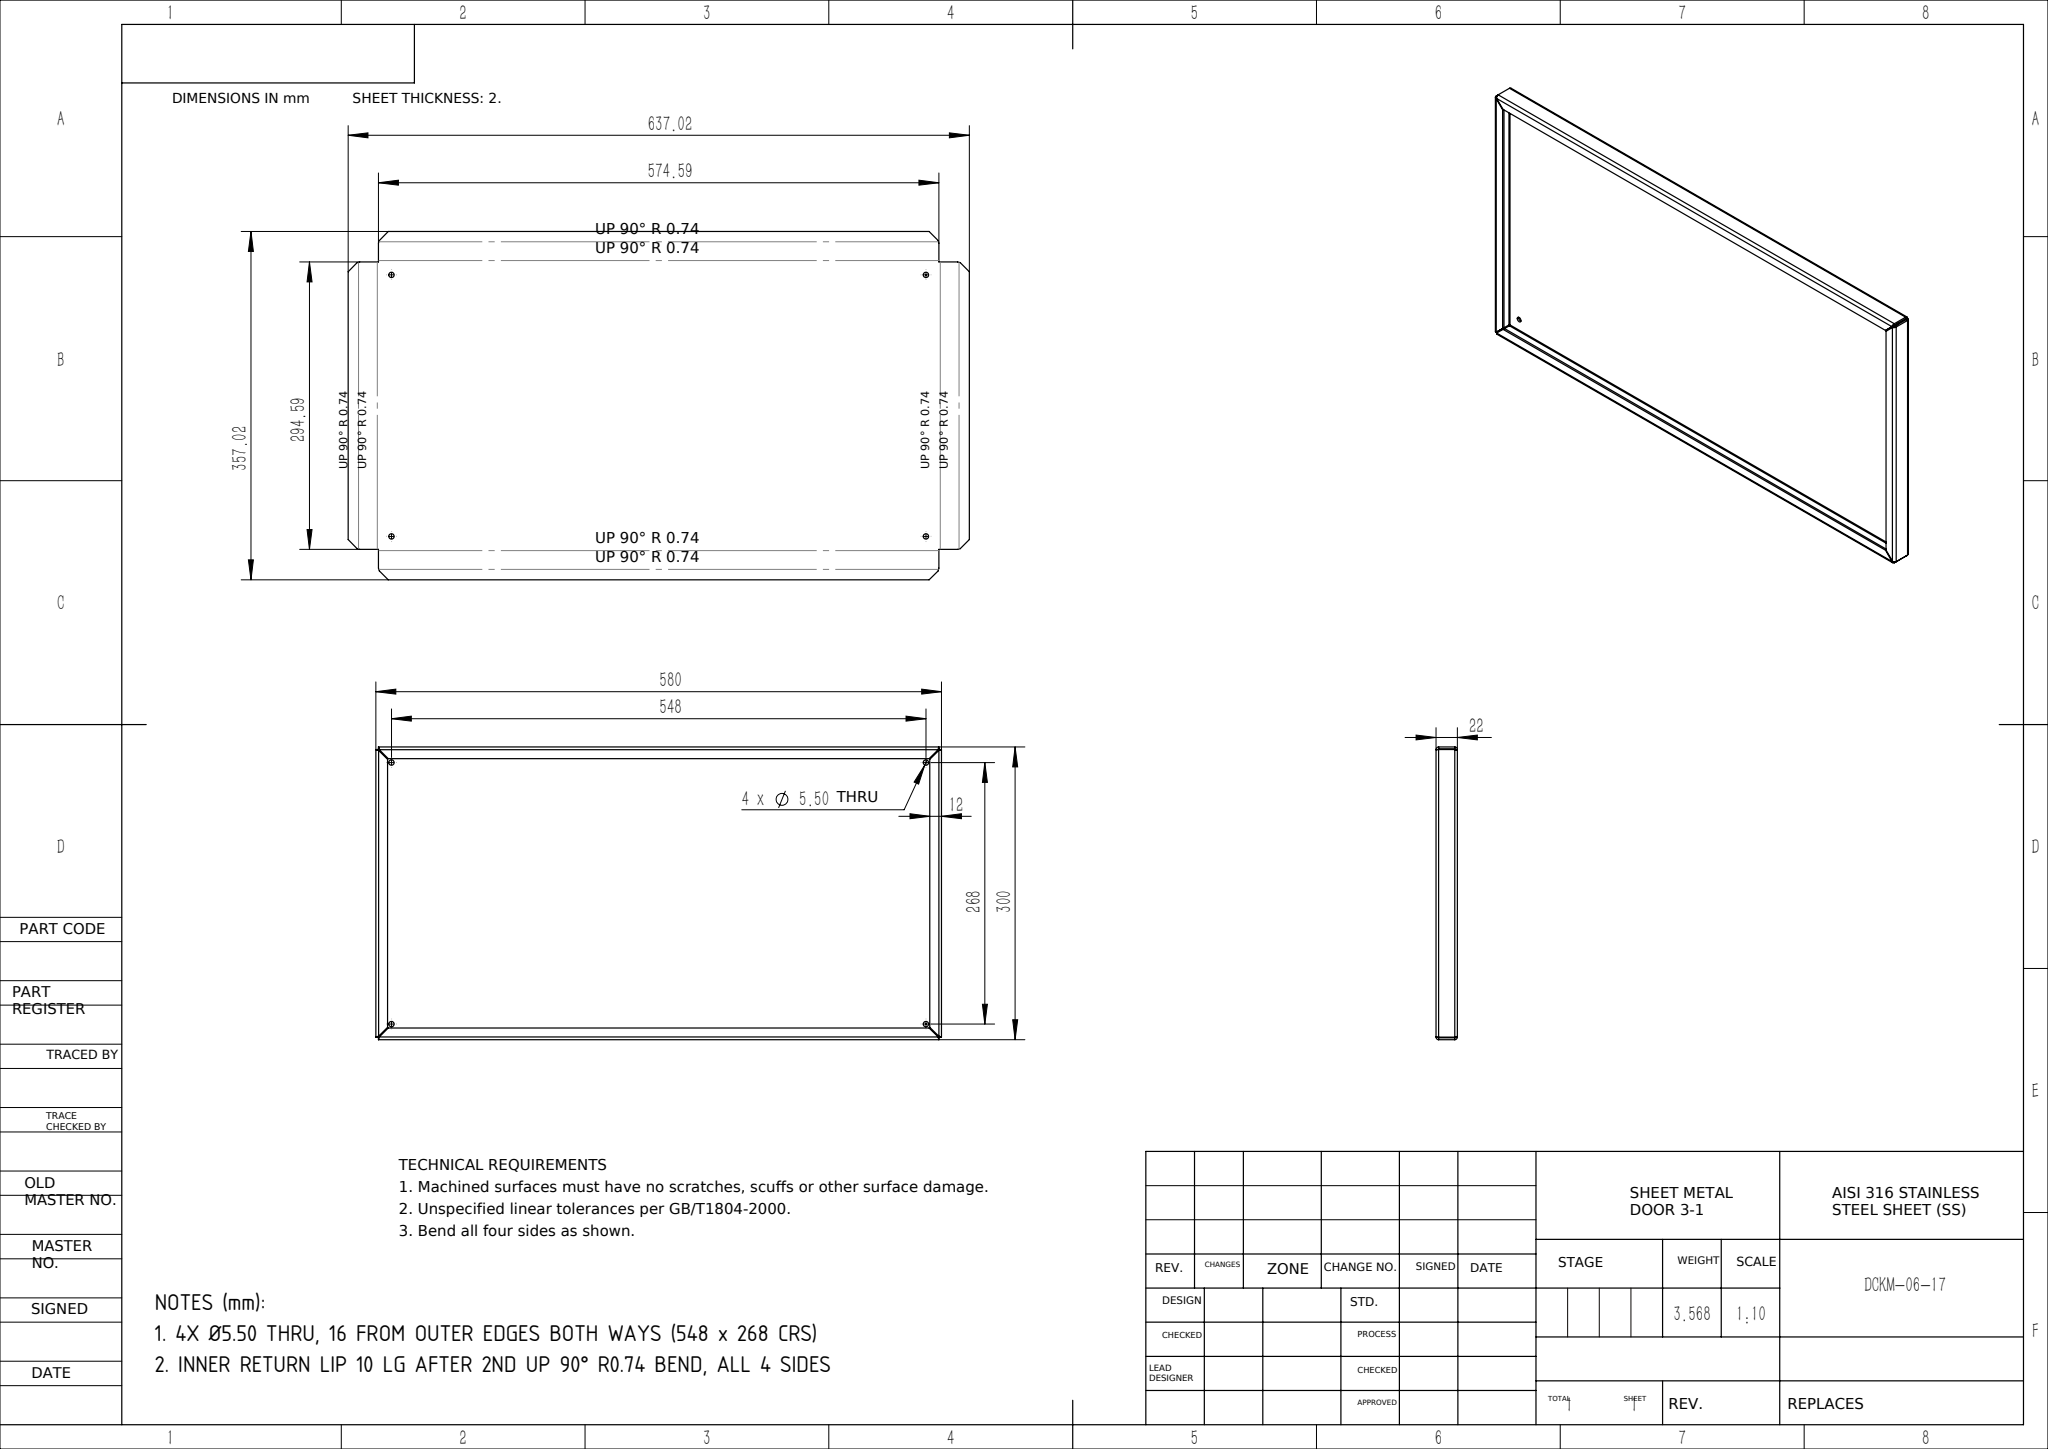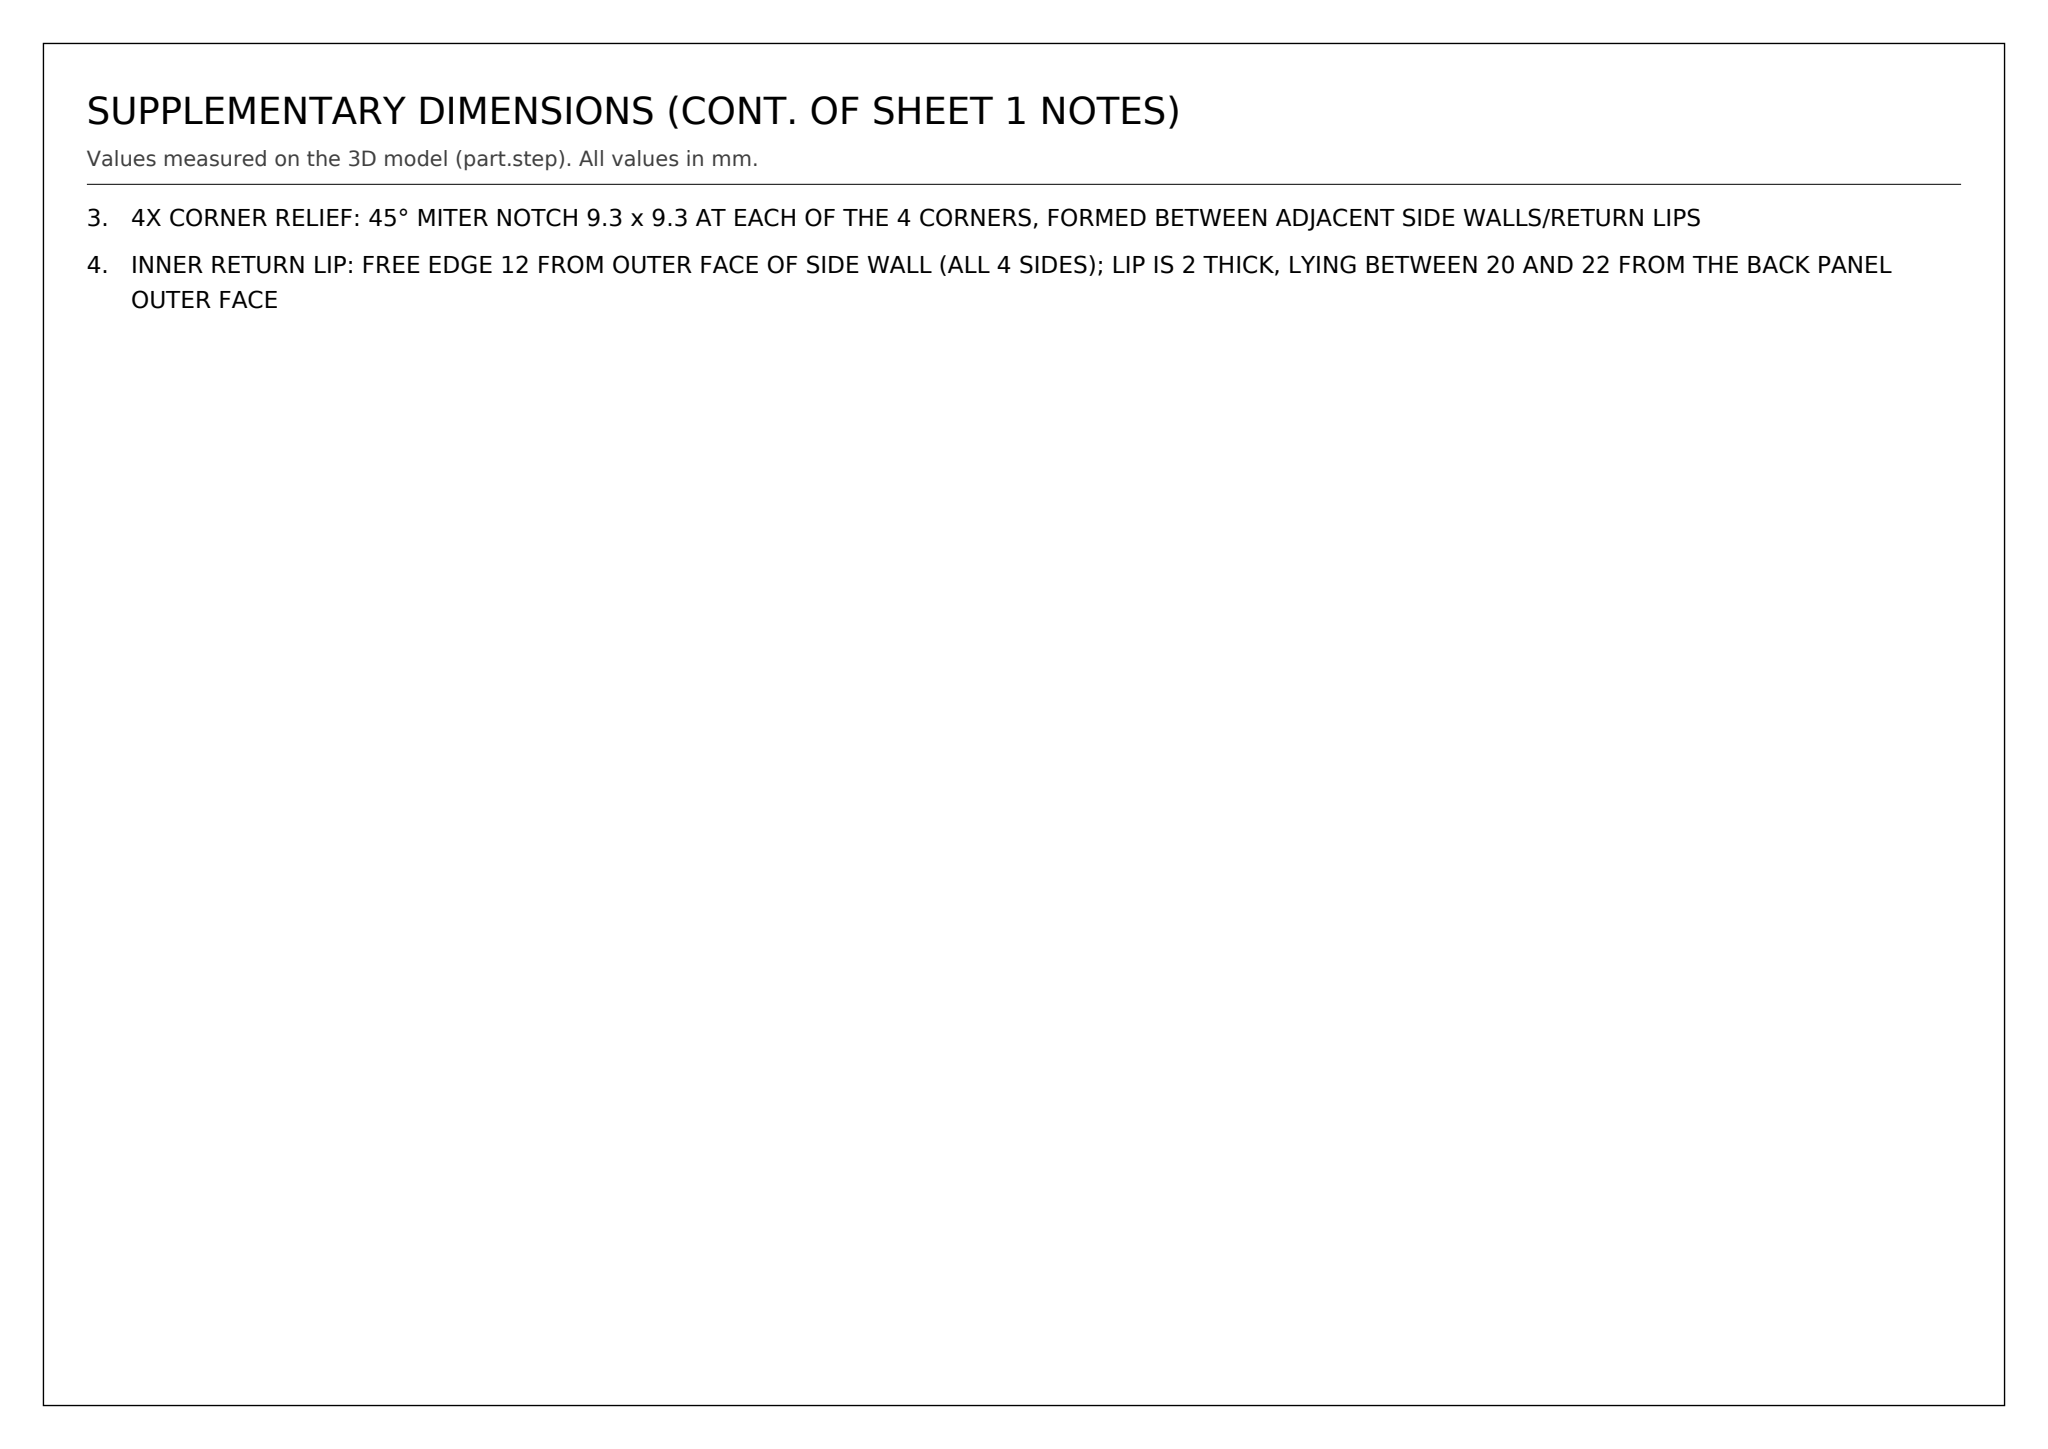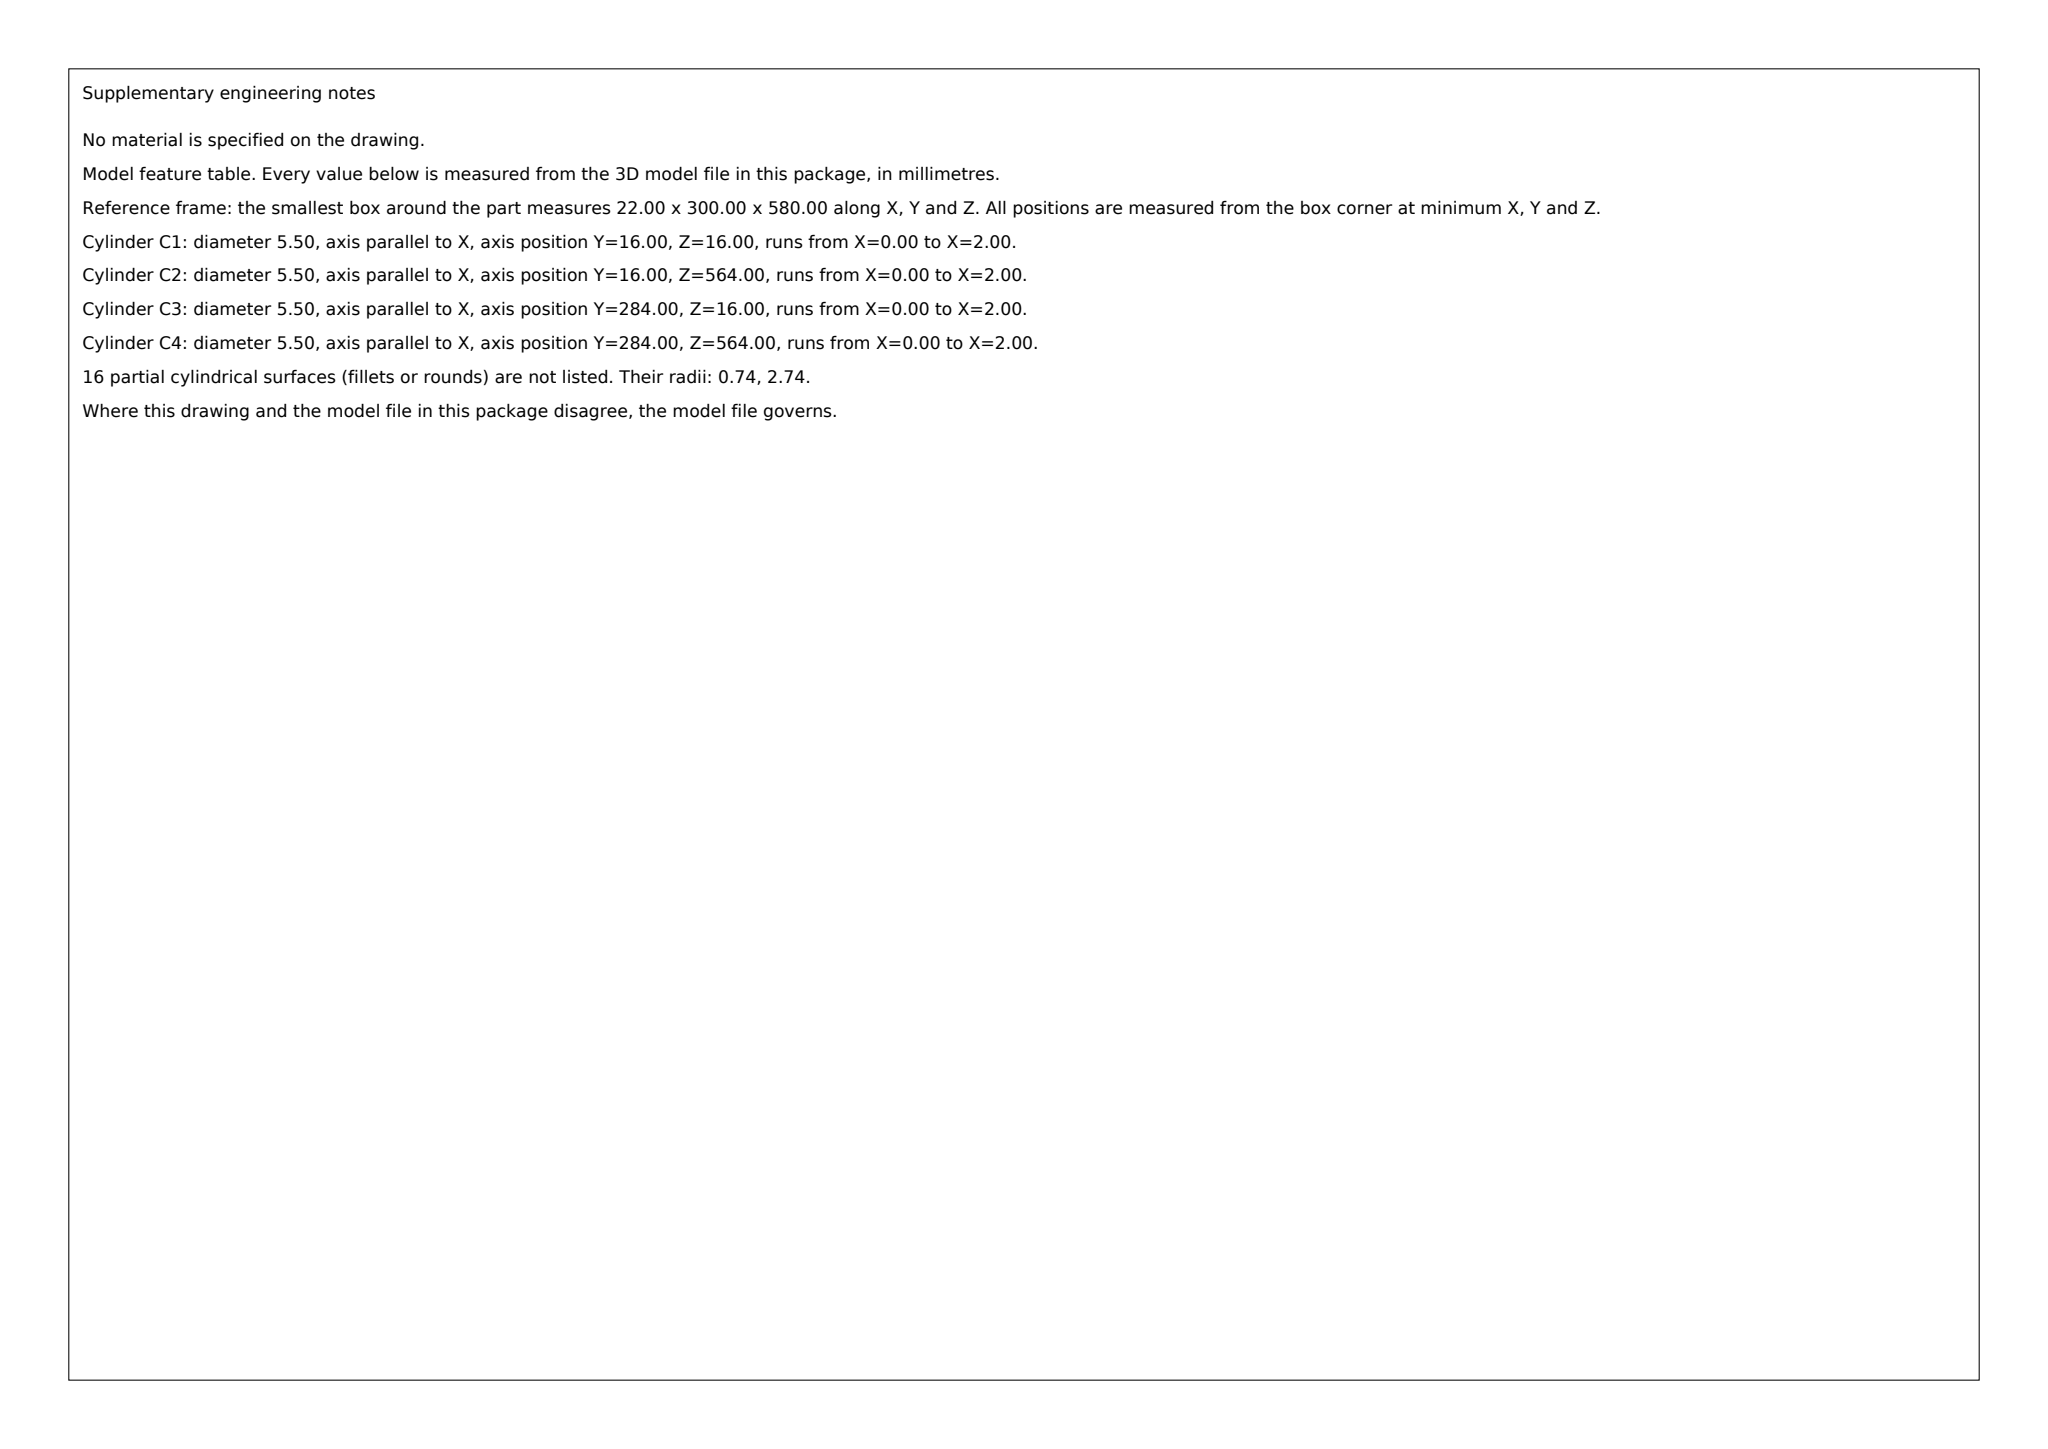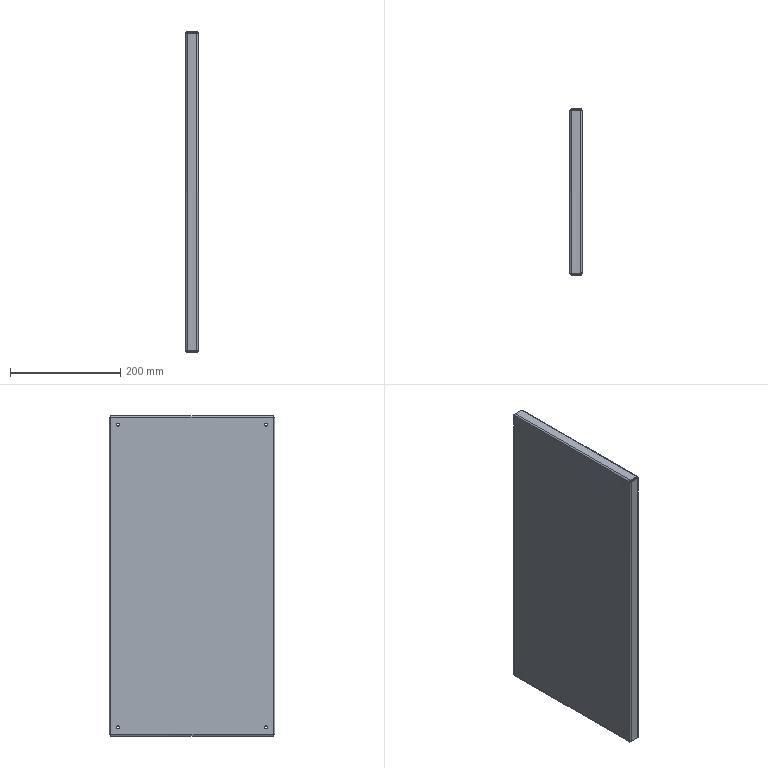Part | SolidWorks | mm | 1 solid | 78 faces | box 22 x 300 x 580 mm | volume 446057 mm3 | plane 38 | cylinder 24 | spline 16 | commonest cylinder face diameters 5.5 x8 5.473 x8 1.473 x8
Drawing notes:
4X Ø5.50 THRU, 16 FROM OUTER EDGES BOTH WAYS (548 x 268 CRS) | from the solid: Ø5.50 x-axis holes at (y,z)=(16.02,16.02),(16.02,564.02),(284.02,16.02),(284.02,564.02); bbox 300.04 x 580.04 -> 16 edge dist, 268 x 548 spacing
INNER RETURN LIP 10 LG AFTER 2ND UP 90° R0.74 BEND, ALL 4 SIDES | from the solid: Lip faces at x=20.02/22.02 span y=2.02-12.02 and z=2.02-12.02 (and 568.02-578.02): 10 mm lip inboard of 2 mm flange wall; 12 dim = 2+10
4X CORNER RELIEF: 45° MITER NOTCH 9.3 x 9.3 AT EACH OF THE 4 CORNERS, FORMED BETWEEN ADJACENT SIDE WALLS/RETURN LIPS | from the solid: inclined_planes: 8 faces at angle_to_xyz_axes [90.0,45.0,45.0], size [2.0,9.3,9.3], bbox_from x=20.0 at the four corners (y 2.8/287.3/288.0/3.5, z 2.8/567.3/568.0/3.5)
INNER RETURN LIP: FREE EDGE 12 FROM OUTER FACE OF SIDE WALL (ALL 4 SIDES); LIP IS 2 THICK, LYING BETWEEN 20 AND 22 FROM THE BACK PANEL OUTER FACE | from the solid: axis_planes: y=12.0 and z=12.0 with x extent [20.0,22.0] (lip inner edge faces); x=20.0 and x=22.0 lip faces, outer walls at y=0.0 / z=0.0